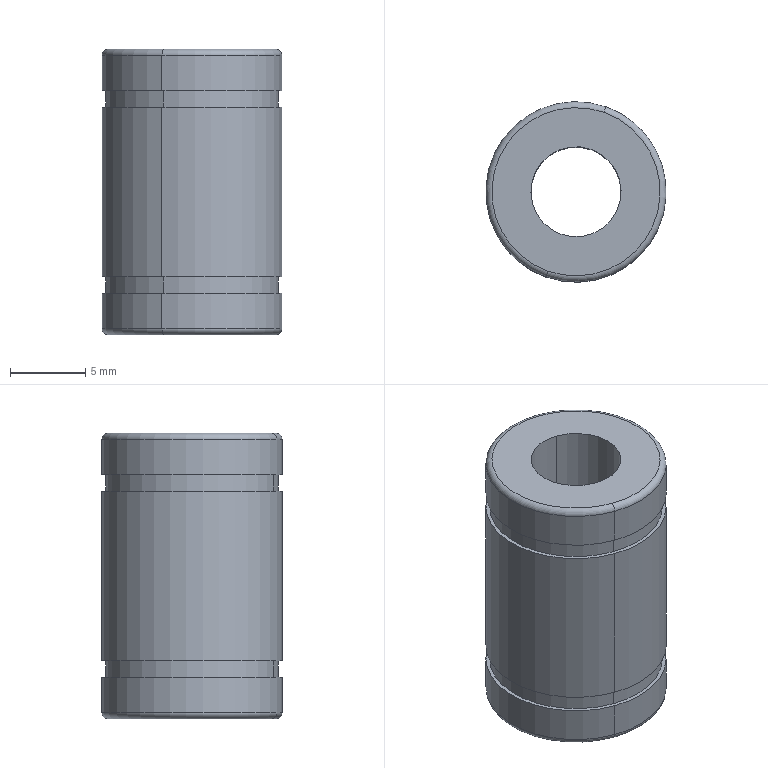Component | SolidWorks | LinearBearingMisumiLMU6-1 | 1 solid | 22 faces | box 12 x 12 x 19 mm | volume 1589 mm3 | cylinder 12 | plane 6 | torus 4 | commonest cylinder face diameters 12 x6 11.5 x4 6 x2 | material 45
build123d program:
from build123d import *


with BuildPart() as part:
    # Sketch1 → Revolve1 (revolve)
    with BuildSketch(Plane.XY, mode=Mode.PRIVATE) as revolve1_sk:
        with BuildLine():
            Line((0, 5.6), (0, 3))
            Line((0, 3), (19, 3))
            Line((19, 3), (19, 5.6))
            ThreePointArc((19, 5.6), (18.883, 5.883), (18.6, 6))
            Line((18.6, 6), (16.25, 6))
            Line((16.25, 6), (16.25, 5.75))
            Line((16.25, 5.75), (15.15, 5.75))
            Line((15.15, 5.75), (15.15, 6))
            Line((15.15, 6), (3.85, 6))
            Line((3.85, 6), (3.85, 5.75))
            Line((3.85, 5.75), (2.75, 5.75))
            Line((2.75, 5.75), (2.75, 6))
            Line((2.75, 6), (0.4, 6))
            ThreePointArc((0.4, 6), (0.1172, 5.883), (0, 5.6))
        make_face()
    revolve(revolve1_sk.sketch.rotate(Axis((19, 0, 0), (-1, 0, 0)), 270), axis=Axis((19, 0, 0), (-1, 0, 0)))


solid = part.part

# Placed as in the assembly
solid = solid.moved(Location((-10, 5.5, 13.5), (0, 90, 0)))
STEP:
#1=COLOUR_RGB('',0.7922,0.8196,0.9333);
#2=FILL_AREA_STYLE_COLOUR('',#1);
#3=FILL_AREA_STYLE('',(#2));
#4=SURFACE_STYLE_FILL_AREA(#3);
#5=SURFACE_SIDE_STYLE('',(#4));
#6=SURFACE_STYLE_USAGE(.BOTH.,#5);
#7=PRESENTATION_STYLE_ASSIGNMENT((#6));
#8=CARTESIAN_POINT('',(-0.315,0.4393,-0.1083));
#9=VERTEX_POINT('',#8);
#10=CARTESIAN_POINT('',(-0.4724,-0.006183,-0.1083));
#11=VERTEX_POINT('',#10);
#12=CARTESIAN_POINT('',(-0.3937,0.2165,-0.1083));
#13=DIRECTION('',(-0.,0.,-1.));
#14=DIRECTION('',(0.3332,0.9428,0.));
#15=AXIS2_PLACEMENT_3D('',#12,#13,#14);
#16=CIRCLE('',#15,0.2362);
#17=EDGE_CURVE('',#9,#11,#16,.T.);
#18=ORIENTED_EDGE('',*,*,#17,.T.);
#19=CARTESIAN_POINT('',(-0.4724,-0.006183,-0.2008));
#20=VERTEX_POINT('',#19);
#21=CARTESIAN_POINT('',(-0.4724,-0.006183,0.5315));
#22=DIRECTION('',(-0.,0.,-1.));
#23=VECTOR('',#22,39.37);
#24=LINE('',#21,#23);
#25=EDGE_CURVE('',#11,#20,#24,.T.);
#26=ORIENTED_EDGE('',*,*,#25,.T.);
#27=CARTESIAN_POINT('',(-0.315,0.4393,-0.2008));
#28=VERTEX_POINT('',#27);
#29=CARTESIAN_POINT('',(-0.3937,0.2165,-0.2008));
#30=DIRECTION('',(-0.,0.,-1.));
#31=DIRECTION('',(0.3332,0.9428,0.));
#32=AXIS2_PLACEMENT_3D('',#29,#30,#31);
#33=CIRCLE('',#32,0.2362);
#34=EDGE_CURVE('',#28,#20,#33,.T.);
#35=ORIENTED_EDGE('',*,*,#34,.F.);
#36=CARTESIAN_POINT('',(-0.315,0.4393,0.5315));
#37=DIRECTION('',(-0.,0.,-1.));
#38=VECTOR('',#37,39.37);
#39=LINE('',#36,#38);
#40=EDGE_CURVE('',#9,#28,#39,.T.);
#41=ORIENTED_EDGE('',*,*,#40,.F.);
#42=EDGE_LOOP('',(#18,#26,#35,#41));
#43=FACE_OUTER_BOUND('',#42,.T.);
#44=CARTESIAN_POINT('',(-0.3937,0.2165,0.5315));
#45=DIRECTION('',(-0.,0.,-1.));
#46=DIRECTION('',(0.3332,0.9428,0.));
#47=AXIS2_PLACEMENT_3D('',#44,#45,#46);
#48=CYLINDRICAL_SURFACE('',#47,0.2362);
#49=ADVANCED_FACE('',(#43),#48,.T.);
#50=CARTESIAN_POINT('',(-0.3183,0.43,-0.06496));
#51=VERTEX_POINT('',#50);
#52=CARTESIAN_POINT('',(-0.4691,0.003097,-0.06496));
#53=VERTEX_POINT('',#52);
#54=CARTESIAN_POINT('',(-0.3937,0.2165,-0.06496));
#55=DIRECTION('',(-0.,0.,-1.));
#56=DIRECTION('',(0.3332,0.9428,0.));
#57=AXIS2_PLACEMENT_3D('',#54,#55,#56);
#58=CIRCLE('',#57,0.2264);
#59=EDGE_CURVE('',#51,#53,#58,.T.);
#60=ORIENTED_EDGE('',*,*,#59,.T.);
#61=CARTESIAN_POINT('',(-0.4691,0.003097,-0.1083));
#62=VERTEX_POINT('',#61);
#63=CARTESIAN_POINT('',(-0.4691,0.003097,0.5315));
#64=DIRECTION('',(-0.,0.,-1.));
#65=VECTOR('',#64,39.37);
#66=LINE('',#63,#65);
#67=EDGE_CURVE('',#53,#62,#66,.T.);
#68=ORIENTED_EDGE('',*,*,#67,.T.);
#69=CARTESIAN_POINT('',(-0.3183,0.43,-0.1083));
#70=VERTEX_POINT('',#69);
#71=CARTESIAN_POINT('',(-0.3937,0.2165,-0.1083));
#72=DIRECTION('',(-0.,0.,-1.));
#73=DIRECTION('',(0.3332,0.9428,0.));
#74=AXIS2_PLACEMENT_3D('',#71,#72,#73);
#75=CIRCLE('',#74,0.2264);
#76=EDGE_CURVE('',#70,#62,#75,.T.);
#77=ORIENTED_EDGE('',*,*,#76,.F.);
#78=CARTESIAN_POINT('',(-0.3183,0.43,0.5315));
#79=DIRECTION('',(-0.,0.,-1.));
#80=VECTOR('',#79,39.37);
#81=LINE('',#78,#80);
#82=EDGE_CURVE('',#51,#70,#81,.T.);
#83=ORIENTED_EDGE('',*,*,#82,.F.);
#84=EDGE_LOOP('',(#60,#68,#77,#83));
#85=FACE_OUTER_BOUND('',#84,.T.);
#86=CARTESIAN_POINT('',(-0.3937,0.2165,0.5315));
#87=DIRECTION('',(-0.,0.,-1.));
#88=DIRECTION('',(0.3332,0.9428,0.));
#89=AXIS2_PLACEMENT_3D('',#86,#87,#88);
#90=CYLINDRICAL_SURFACE('',#89,0.2264);
#91=ADVANCED_FACE('',(#85),#90,.T.);
#92=CARTESIAN_POINT('',(-0.315,0.4393,0.3799));
#93=VERTEX_POINT('',#92);
#94=CARTESIAN_POINT('',(-0.4724,-0.006183,0.3799));
#95=VERTEX_POINT('',#94);
#96=CARTESIAN_POINT('',(-0.3937,0.2165,0.3799));
#97=DIRECTION('',(-0.,0.,-1.));
#98=DIRECTION('',(0.3332,0.9428,0.));
#99=AXIS2_PLACEMENT_3D('',#96,#97,#98);
#100=CIRCLE('',#99,0.2362);
#101=EDGE_CURVE('',#93,#95,#100,.T.);
#102=ORIENTED_EDGE('',*,*,#101,.T.);
#103=CARTESIAN_POINT('',(-0.4724,-0.006183,-0.06496));
#104=VERTEX_POINT('',#103);
#105=CARTESIAN_POINT('',(-0.4724,-0.006183,0.5315));
#106=DIRECTION('',(-0.,0.,-1.));
#107=VECTOR('',#106,39.37);
#108=LINE('',#105,#107);
#109=EDGE_CURVE('',#95,#104,#108,.T.);
#110=ORIENTED_EDGE('',*,*,#109,.T.);
#111=CARTESIAN_POINT('',(-0.315,0.4393,-0.06496));
#112=VERTEX_POINT('',#111);
#113=CARTESIAN_POINT('',(-0.3937,0.2165,-0.06496));
#114=DIRECTION('',(-0.,0.,-1.));
#115=DIRECTION('',(0.3332,0.9428,0.));
#116=AXIS2_PLACEMENT_3D('',#113,#114,#115);
#117=CIRCLE('',#116,0.2362);
#118=EDGE_CURVE('',#112,#104,#117,.T.);
#119=ORIENTED_EDGE('',*,*,#118,.F.);
#120=CARTESIAN_POINT('',(-0.315,0.4393,0.5315));
#121=DIRECTION('',(-0.,0.,-1.));
#122=VECTOR('',#121,39.37);
#123=LINE('',#120,#122);
#124=EDGE_CURVE('',#93,#112,#123,.T.);
#125=ORIENTED_EDGE('',*,*,#124,.F.);
#126=EDGE_LOOP('',(#102,#110,#119,#125));
#127=FACE_OUTER_BOUND('',#126,.T.);
#128=CARTESIAN_POINT('',(-0.3937,0.2165,0.5315));
#129=DIRECTION('',(-0.,0.,-1.));
#130=DIRECTION('',(0.3332,0.9428,0.));
#131=AXIS2_PLACEMENT_3D('',#128,#129,#130);
#132=CYLINDRICAL_SURFACE('',#131,0.2362);
#133=ADVANCED_FACE('',(#127),#132,.T.);
#134=CARTESIAN_POINT('',(-0.3183,0.43,0.4232));
#135=VERTEX_POINT('',#134);
#136=CARTESIAN_POINT('',(-0.4691,0.003097,0.4232));
#137=VERTEX_POINT('',#136);
#138=CARTESIAN_POINT('',(-0.3937,0.2165,0.4232));
#139=DIRECTION('',(-0.,0.,-1.));
#140=DIRECTION('',(0.3332,0.9428,0.));
#141=AXIS2_PLACEMENT_3D('',#138,#139,#140);
#142=CIRCLE('',#141,0.2264);
#143=EDGE_CURVE('',#135,#137,#142,.T.);
#144=ORIENTED_EDGE('',*,*,#143,.T.);
#145=CARTESIAN_POINT('',(-0.4691,0.003097,0.3799));
#146=VERTEX_POINT('',#145);
#147=CARTESIAN_POINT('',(-0.4691,0.003097,0.5315));
#148=DIRECTION('',(-0.,0.,-1.));
#149=VECTOR('',#148,39.37);
#150=LINE('',#147,#149);
#151=EDGE_CURVE('',#137,#146,#150,.T.);
#152=ORIENTED_EDGE('',*,*,#151,.T.);
#153=CARTESIAN_POINT('',(-0.3183,0.43,0.3799));
#154=VERTEX_POINT('',#153);
#155=CARTESIAN_POINT('',(-0.3937,0.2165,0.3799));
#156=DIRECTION('',(-0.,0.,-1.));
#157=DIRECTION('',(0.3332,0.9428,0.));
#158=AXIS2_PLACEMENT_3D('',#155,#156,#157);
#159=CIRCLE('',#158,0.2264);
#160=EDGE_CURVE('',#154,#146,#159,.T.);
#161=ORIENTED_EDGE('',*,*,#160,.F.);
#162=CARTESIAN_POINT('',(-0.3183,0.43,0.5315));
#163=DIRECTION('',(-0.,0.,-1.));
#164=VECTOR('',#163,39.37);
#165=LINE('',#162,#164);
#166=EDGE_CURVE('',#135,#154,#165,.T.);
#167=ORIENTED_EDGE('',*,*,#166,.F.);
#168=EDGE_LOOP('',(#144,#152,#161,#167));
#169=FACE_OUTER_BOUND('',#168,.T.);
#170=CARTESIAN_POINT('',(-0.3937,0.2165,0.5315));
#171=DIRECTION('',(-0.,0.,-1.));
#172=DIRECTION('',(0.3332,0.9428,0.));
#173=AXIS2_PLACEMENT_3D('',#170,#171,#172);
#174=CYLINDRICAL_SURFACE('',#173,0.2264);
#175=ADVANCED_FACE('',(#169),#174,.T.);
#176=CARTESIAN_POINT('',(-0.315,0.4393,0.5157));
#177=VERTEX_POINT('',#176);
#178=CARTESIAN_POINT('',(-0.4724,-0.006183,0.5157));
#179=VERTEX_POINT('',#178);
#180=CARTESIAN_POINT('',(-0.3937,0.2165,0.5157));
#181=DIRECTION('',(-0.,0.,-1.));
#182=DIRECTION('',(0.3332,0.9428,0.));
#183=AXIS2_PLACEMENT_3D('',#180,#181,#182);
#184=CIRCLE('',#183,0.2362);
#185=EDGE_CURVE('',#177,#179,#184,.T.);
#186=ORIENTED_EDGE('',*,*,#185,.T.);
#187=CARTESIAN_POINT('',(-0.4724,-0.006183,0.4232));
#188=VERTEX_POINT('',#187);
#189=CARTESIAN_POINT('',(-0.4724,-0.006183,0.5315));
#190=DIRECTION('',(-0.,0.,-1.));
#191=VECTOR('',#190,39.37);
#192=LINE('',#189,#191);
#193=EDGE_CURVE('',#179,#188,#192,.T.);
#194=ORIENTED_EDGE('',*,*,#193,.T.);
#195=CARTESIAN_POINT('',(-0.315,0.4393,0.4232));
#196=VERTEX_POINT('',#195);
#197=CARTESIAN_POINT('',(-0.3937,0.2165,0.4232));
#198=DIRECTION('',(-0.,0.,-1.));
#199=DIRECTION('',(0.3332,0.9428,0.));
#200=AXIS2_PLACEMENT_3D('',#197,#198,#199);
#201=CIRCLE('',#200,0.2362);
#202=EDGE_CURVE('',#196,#188,#201,.T.);
#203=ORIENTED_EDGE('',*,*,#202,.F.);
#204=CARTESIAN_POINT('',(-0.315,0.4393,0.5315));
#205=DIRECTION('',(-0.,0.,-1.));
#206=VECTOR('',#205,39.37);
#207=LINE('',#204,#206);
#208=EDGE_CURVE('',#177,#196,#207,.T.);
#209=ORIENTED_EDGE('',*,*,#208,.F.);
#210=EDGE_LOOP('',(#186,#194,#203,#209));
#211=FACE_OUTER_BOUND('',#210,.T.);
#212=CARTESIAN_POINT('',(-0.3937,0.2165,0.5315));
#213=DIRECTION('',(-0.,0.,-1.));
#214=DIRECTION('',(0.3332,0.9428,0.));
#215=AXIS2_PLACEMENT_3D('',#212,#213,#214);
#216=CYLINDRICAL_SURFACE('',#215,0.2362);
#217=ADVANCED_FACE('',(#211),#216,.T.);
#218=CARTESIAN_POINT('',(-0.3202,0.4244,0.5315));
#219=VERTEX_POINT('',#218);
#220=CARTESIAN_POINT('',(-0.4672,0.008665,0.5315));
#221=VERTEX_POINT('',#220);
#222=CARTESIAN_POINT('',(-0.3937,0.2165,0.5315));
#223=DIRECTION('',(-0.,0.,-1.));
#224=DIRECTION('',(0.3332,0.9428,0.));
#225=AXIS2_PLACEMENT_3D('',#222,#223,#224);
#226=CIRCLE('',#225,0.2205);
#227=EDGE_CURVE('',#219,#221,#226,.T.);
#228=ORIENTED_EDGE('',*,*,#227,.T.);
#229=CARTESIAN_POINT('',(-0.4672,0.008665,0.5157));
#230=DIRECTION('',(0.9428,-0.3332,-0.));
#231=DIRECTION('',(0.3332,0.9428,0.));
#232=AXIS2_PLACEMENT_3D('',#229,#230,#231);
#233=CIRCLE('',#232,0.01575);
#234=EDGE_CURVE('',#221,#179,#233,.T.);
#235=ORIENTED_EDGE('',*,*,#234,.T.);
#236=ORIENTED_EDGE('',*,*,#185,.F.);
#237=CARTESIAN_POINT('',(-0.3202,0.4244,0.5157));
#238=DIRECTION('',(-0.9428,0.3332,0.));
#239=DIRECTION('',(-0.3332,-0.9428,0.));
#240=AXIS2_PLACEMENT_3D('',#237,#238,#239);
#241=CIRCLE('',#240,0.01575);
#242=EDGE_CURVE('',#219,#177,#241,.T.);
#243=ORIENTED_EDGE('',*,*,#242,.F.);
#244=EDGE_LOOP('',(#228,#235,#236,#243));
#245=FACE_OUTER_BOUND('',#244,.T.);
#246=CARTESIAN_POINT('',(-0.3937,0.2165,0.5157));
#247=DIRECTION('',(-0.,0.,-1.));
#248=DIRECTION('',(0.3332,0.9428,0.));
#249=AXIS2_PLACEMENT_3D('',#246,#247,#248);
#250=TOROIDAL_SURFACE('',#249,0.2205,0.01575);
#251=ADVANCED_FACE('',(#245),#250,.T.);
#252=CARTESIAN_POINT('',(-0.4331,0.1052,0.5315));
#253=VERTEX_POINT('',#252);
#254=CARTESIAN_POINT('',(-0.3543,0.3279,0.5315));
#255=VERTEX_POINT('',#254);
#256=CARTESIAN_POINT('',(-0.3937,0.2165,0.5315));
#257=DIRECTION('',(-0.,0.,-1.));
#258=DIRECTION('',(0.3332,0.9428,0.));
#259=AXIS2_PLACEMENT_3D('',#256,#257,#258);
#260=CIRCLE('',#259,0.1181);
#261=EDGE_CURVE('',#253,#255,#260,.T.);
#262=ORIENTED_EDGE('',*,*,#261,.F.);
#263=CARTESIAN_POINT('',(-0.4331,0.1052,-0.2165));
#264=VERTEX_POINT('',#263);
#265=CARTESIAN_POINT('',(-0.4331,0.1052,0.5315));
#266=DIRECTION('',(-0.,0.,-1.));
#267=VECTOR('',#266,39.37);
#268=LINE('',#265,#267);
#269=EDGE_CURVE('',#253,#264,#268,.T.);
#270=ORIENTED_EDGE('',*,*,#269,.T.);
#271=CARTESIAN_POINT('',(-0.3543,0.3279,-0.2165));
#272=VERTEX_POINT('',#271);
#273=CARTESIAN_POINT('',(-0.3937,0.2165,-0.2165));
#274=DIRECTION('',(-0.,0.,-1.));
#275=DIRECTION('',(0.3332,0.9428,0.));
#276=AXIS2_PLACEMENT_3D('',#273,#274,#275);
#277=CIRCLE('',#276,0.1181);
#278=EDGE_CURVE('',#264,#272,#277,.T.);
#279=ORIENTED_EDGE('',*,*,#278,.T.);
#280=CARTESIAN_POINT('',(-0.3543,0.3279,0.5315));
#281=DIRECTION('',(-0.,0.,-1.));
#282=VECTOR('',#281,39.37);
#283=LINE('',#280,#282);
#284=EDGE_CURVE('',#255,#272,#283,.T.);
#285=ORIENTED_EDGE('',*,*,#284,.F.);
#286=EDGE_LOOP('',(#262,#270,#279,#285));
#287=FACE_OUTER_BOUND('',#286,.T.);
#288=CARTESIAN_POINT('',(-0.3937,0.2165,0.5315));
#289=DIRECTION('',(-0.,0.,-1.));
#290=DIRECTION('',(0.3332,0.9428,0.));
#291=AXIS2_PLACEMENT_3D('',#288,#289,#290);
#292=CYLINDRICAL_SURFACE('',#291,0.1181);
#293=ADVANCED_FACE('',(#287),#292,.F.);
#294=ORIENTED_EDGE('',*,*,#34,.T.);
#295=CARTESIAN_POINT('',(-0.4672,0.008665,-0.2165));
#296=VERTEX_POINT('',#295);
#297=CARTESIAN_POINT('',(-0.4672,0.008665,-0.2008));
#298=DIRECTION('',(0.9428,-0.3332,-0.));
#299=DIRECTION('',(0.3332,0.9428,0.));
#300=AXIS2_PLACEMENT_3D('',#297,#298,#299);
#301=CIRCLE('',#300,0.01575);
#302=EDGE_CURVE('',#20,#296,#301,.T.);
#303=ORIENTED_EDGE('',*,*,#302,.T.);
#304=CARTESIAN_POINT('',(-0.3202,0.4244,-0.2165));
#305=VERTEX_POINT('',#304);
#306=CARTESIAN_POINT('',(-0.3937,0.2165,-0.2165));
#307=DIRECTION('',(-0.,0.,-1.));
#308=DIRECTION('',(0.3332,0.9428,0.));
#309=AXIS2_PLACEMENT_3D('',#306,#307,#308);
#310=CIRCLE('',#309,0.2205);
#311=EDGE_CURVE('',#305,#296,#310,.T.);
#312=ORIENTED_EDGE('',*,*,#311,.F.);
#313=CARTESIAN_POINT('',(-0.3202,0.4244,-0.2008));
#314=DIRECTION('',(-0.9428,0.3332,0.));
#315=DIRECTION('',(-0.3332,-0.9428,0.));
#316=AXIS2_PLACEMENT_3D('',#313,#314,#315);
#317=CIRCLE('',#316,0.01575);
#318=EDGE_CURVE('',#28,#305,#317,.T.);
#319=ORIENTED_EDGE('',*,*,#318,.F.);
#320=EDGE_LOOP('',(#294,#303,#312,#319));
#321=FACE_OUTER_BOUND('',#320,.T.);
#322=CARTESIAN_POINT('',(-0.3937,0.2165,-0.2008));
#323=DIRECTION('',(-0.,0.,-1.));
#324=DIRECTION('',(0.3332,0.9428,0.));
#325=AXIS2_PLACEMENT_3D('',#322,#323,#324);
#326=TOROIDAL_SURFACE('',#325,0.2205,0.01575);
#327=ADVANCED_FACE('',(#321),#326,.T.);
#328=ORIENTED_EDGE('',*,*,#302,.F.);
#329=CARTESIAN_POINT('',(-0.3937,0.2165,-0.2008));
#330=DIRECTION('',(-0.,0.,-1.));
#331=DIRECTION('',(0.3332,0.9428,0.));
#332=AXIS2_PLACEMENT_3D('',#329,#330,#331);
#333=CIRCLE('',#332,0.2362);
#334=EDGE_CURVE('',#20,#28,#333,.T.);
#335=ORIENTED_EDGE('',*,*,#334,.T.);
#336=ORIENTED_EDGE('',*,*,#318,.T.);
#337=CARTESIAN_POINT('',(-0.3937,0.2165,-0.2165));
#338=DIRECTION('',(-0.,0.,-1.));
#339=DIRECTION('',(0.3332,0.9428,0.));
#340=AXIS2_PLACEMENT_3D('',#337,#338,#339);
#341=CIRCLE('',#340,0.2205);
#342=EDGE_CURVE('',#296,#305,#341,.T.);
#343=ORIENTED_EDGE('',*,*,#342,.F.);
#344=EDGE_LOOP('',(#328,#335,#336,#343));
#345=FACE_OUTER_BOUND('',#344,.T.);
#346=CARTESIAN_POINT('',(-0.3937,0.2165,-0.2008));
#347=DIRECTION('',(-0.,0.,-1.));
#348=DIRECTION('',(0.3332,0.9428,0.));
#349=AXIS2_PLACEMENT_3D('',#346,#347,#348);
#350=TOROIDAL_SURFACE('',#349,0.2205,0.01575);
#351=ADVANCED_FACE('',(#345),#350,.T.);
#352=CARTESIAN_POINT('',(-0.3937,0.2165,-0.2165));
#353=DIRECTION('',(-0.,0.,-1.));
#354=DIRECTION('',(0.3332,0.9428,0.));
#355=AXIS2_PLACEMENT_3D('',#352,#353,#354);
#356=CIRCLE('',#355,0.1181);
#357=EDGE_CURVE('',#272,#264,#356,.T.);
#358=ORIENTED_EDGE('',*,*,#357,.F.);
#359=ORIENTED_EDGE('',*,*,#278,.F.);
#360=EDGE_LOOP('',(#358,#359));
#361=FACE_BOUND('',#360,.T.);
#362=ORIENTED_EDGE('',*,*,#311,.T.);
#363=ORIENTED_EDGE('',*,*,#342,.T.);
#364=EDGE_LOOP('',(#362,#363));
#365=FACE_OUTER_BOUND('',#364,.T.);
#366=CARTESIAN_POINT('',(-0.1858,0.1431,-0.2165));
#367=DIRECTION('',(0.,-0.,1.));
#368=DIRECTION('',(-0.3332,-0.9428,-0.));
#369=AXIS2_PLACEMENT_3D('',#366,#367,#368);
#370=PLANE('',#369);
#371=ADVANCED_FACE('',(#361,#365),#370,.F.);
#372=ORIENTED_EDGE('',*,*,#269,.F.);
#373=CARTESIAN_POINT('',(-0.3937,0.2165,0.5315));
#374=DIRECTION('',(-0.,0.,-1.));
#375=DIRECTION('',(0.3332,0.9428,0.));
#376=AXIS2_PLACEMENT_3D('',#373,#374,#375);
#377=CIRCLE('',#376,0.1181);
#378=EDGE_CURVE('',#255,#253,#377,.T.);
#379=ORIENTED_EDGE('',*,*,#378,.F.);
#380=ORIENTED_EDGE('',*,*,#284,.T.);
#381=ORIENTED_EDGE('',*,*,#357,.T.);
#382=EDGE_LOOP('',(#372,#379,#380,#381));
#383=FACE_OUTER_BOUND('',#382,.T.);
#384=CARTESIAN_POINT('',(-0.3937,0.2165,0.5315));
#385=DIRECTION('',(-0.,0.,-1.));
#386=DIRECTION('',(0.3332,0.9428,0.));
#387=AXIS2_PLACEMENT_3D('',#384,#385,#386);
#388=CYLINDRICAL_SURFACE('',#387,0.1181);
#389=ADVANCED_FACE('',(#383),#388,.F.);
#390=ORIENTED_EDGE('',*,*,#227,.F.);
#391=CARTESIAN_POINT('',(-0.3937,0.2165,0.5315));
#392=DIRECTION('',(-0.,0.,-1.));
#393=DIRECTION('',(0.3332,0.9428,0.));
#394=AXIS2_PLACEMENT_3D('',#391,#392,#393);
#395=CIRCLE('',#394,0.2205);
#396=EDGE_CURVE('',#221,#219,#395,.T.);
#397=ORIENTED_EDGE('',*,*,#396,.F.);
#398=EDGE_LOOP('',(#390,#397));
#399=FACE_OUTER_BOUND('',#398,.T.);
#400=ORIENTED_EDGE('',*,*,#378,.T.);
#401=ORIENTED_EDGE('',*,*,#261,.T.);
#402=EDGE_LOOP('',(#400,#401));
#403=FACE_BOUND('',#402,.T.);
#404=CARTESIAN_POINT('',(-0.2823,0.1772,0.5315));
#405=DIRECTION('',(-0.,0.,-1.));
#406=DIRECTION('',(0.3332,0.9428,0.));
#407=AXIS2_PLACEMENT_3D('',#404,#405,#406);
#408=PLANE('',#407);
#409=ADVANCED_FACE('',(#399,#403),#408,.F.);
#410=ORIENTED_EDGE('',*,*,#234,.F.);
#411=ORIENTED_EDGE('',*,*,#396,.T.);
#412=ORIENTED_EDGE('',*,*,#242,.T.);
#413=CARTESIAN_POINT('',(-0.3937,0.2165,0.5157));
#414=DIRECTION('',(-0.,0.,-1.));
#415=DIRECTION('',(0.3332,0.9428,0.));
#416=AXIS2_PLACEMENT_3D('',#413,#414,#415);
#417=CIRCLE('',#416,0.2362);
#418=EDGE_CURVE('',#179,#177,#417,.T.);
#419=ORIENTED_EDGE('',*,*,#418,.F.);
#420=EDGE_LOOP('',(#410,#411,#412,#419));
#421=FACE_OUTER_BOUND('',#420,.T.);
#422=CARTESIAN_POINT('',(-0.3937,0.2165,0.5157));
#423=DIRECTION('',(-0.,0.,-1.));
#424=DIRECTION('',(0.3332,0.9428,0.));
#425=AXIS2_PLACEMENT_3D('',#422,#423,#424);
#426=TOROIDAL_SURFACE('',#425,0.2205,0.01575);
#427=ADVANCED_FACE('',(#421),#426,.T.);
#428=ORIENTED_EDGE('',*,*,#193,.F.);
#429=ORIENTED_EDGE('',*,*,#418,.T.);
#430=ORIENTED_EDGE('',*,*,#208,.T.);
#431=CARTESIAN_POINT('',(-0.3937,0.2165,0.4232));
#432=DIRECTION('',(-0.,0.,-1.));
#433=DIRECTION('',(0.3332,0.9428,0.));
#434=AXIS2_PLACEMENT_3D('',#431,#432,#433);
#435=CIRCLE('',#434,0.2362);
#436=EDGE_CURVE('',#188,#196,#435,.T.);
#437=ORIENTED_EDGE('',*,*,#436,.F.);
#438=EDGE_LOOP('',(#428,#429,#430,#437));
#439=FACE_OUTER_BOUND('',#438,.T.);
#440=CARTESIAN_POINT('',(-0.3937,0.2165,0.5315));
#441=DIRECTION('',(-0.,0.,-1.));
#442=DIRECTION('',(0.3332,0.9428,0.));
#443=AXIS2_PLACEMENT_3D('',#440,#441,#442);
#444=CYLINDRICAL_SURFACE('',#443,0.2362);
#445=ADVANCED_FACE('',(#439),#444,.T.);
#446=ORIENTED_EDGE('',*,*,#143,.F.);
#447=CARTESIAN_POINT('',(-0.3937,0.2165,0.4232));
#448=DIRECTION('',(-0.,0.,-1.));
#449=DIRECTION('',(0.3332,0.9428,0.));
#450=AXIS2_PLACEMENT_3D('',#447,#448,#449);
#451=CIRCLE('',#450,0.2264);
#452=EDGE_CURVE('',#137,#135,#451,.T.);
#453=ORIENTED_EDGE('',*,*,#452,.F.);
#454=EDGE_LOOP('',(#446,#453));
#455=FACE_BOUND('',#454,.T.);
#456=ORIENTED_EDGE('',*,*,#202,.T.);
#457=ORIENTED_EDGE('',*,*,#436,.T.);
#458=EDGE_LOOP('',(#456,#457));
#459=FACE_OUTER_BOUND('',#458,.T.);
#460=CARTESIAN_POINT('',(-0.171,0.1378,0.4232));
#461=DIRECTION('',(0.,-0.,1.));
#462=DIRECTION('',(-0.3332,-0.9428,-0.));
#463=AXIS2_PLACEMENT_3D('',#460,#461,#462);
#464=PLANE('',#463);
#465=ADVANCED_FACE('',(#455,#459),#464,.F.);
#466=ORIENTED_EDGE('',*,*,#151,.F.);
#467=ORIENTED_EDGE('',*,*,#452,.T.);
#468=ORIENTED_EDGE('',*,*,#166,.T.);
#469=CARTESIAN_POINT('',(-0.3937,0.2165,0.3799));
#470=DIRECTION('',(-0.,0.,-1.));
#471=DIRECTION('',(0.3332,0.9428,0.));
#472=AXIS2_PLACEMENT_3D('',#469,#470,#471);
#473=CIRCLE('',#472,0.2264);
#474=EDGE_CURVE('',#146,#154,#473,.T.);
#475=ORIENTED_EDGE('',*,*,#474,.F.);
#476=EDGE_LOOP('',(#466,#467,#468,#475));
#477=FACE_OUTER_BOUND('',#476,.T.);
#478=CARTESIAN_POINT('',(-0.3937,0.2165,0.5315));
#479=DIRECTION('',(-0.,0.,-1.));
#480=DIRECTION('',(0.3332,0.9428,0.));
#481=AXIS2_PLACEMENT_3D('',#478,#479,#480);
#482=CYLINDRICAL_SURFACE('',#481,0.2264);
#483=ADVANCED_FACE('',(#477),#482,.T.);
#484=ORIENTED_EDGE('',*,*,#101,.F.);
#485=CARTESIAN_POINT('',(-0.3937,0.2165,0.3799));
#486=DIRECTION('',(-0.,0.,-1.));
#487=DIRECTION('',(0.3332,0.9428,0.));
#488=AXIS2_PLACEMENT_3D('',#485,#486,#487);
#489=CIRCLE('',#488,0.2362);
#490=EDGE_CURVE('',#95,#93,#489,.T.);
#491=ORIENTED_EDGE('',*,*,#490,.F.);
#492=EDGE_LOOP('',(#484,#491));
#493=FACE_OUTER_BOUND('',#492,.T.);
#494=ORIENTED_EDGE('',*,*,#160,.T.);
#495=ORIENTED_EDGE('',*,*,#474,.T.);
#496=EDGE_LOOP('',(#494,#495));
#497=FACE_BOUND('',#496,.T.);
#498=CARTESIAN_POINT('',(-0.1803,0.1411,0.3799));
#499=DIRECTION('',(-0.,0.,-1.));
#500=DIRECTION('',(0.3332,0.9428,0.));
#501=AXIS2_PLACEMENT_3D('',#498,#499,#500);
#502=PLANE('',#501);
#503=ADVANCED_FACE('',(#493,#497),#502,.F.);
#504=ORIENTED_EDGE('',*,*,#109,.F.);
#505=ORIENTED_EDGE('',*,*,#490,.T.);
#506=ORIENTED_EDGE('',*,*,#124,.T.);
#507=CARTESIAN_POINT('',(-0.3937,0.2165,-0.06496));
#508=DIRECTION('',(-0.,0.,-1.));
#509=DIRECTION('',(0.3332,0.9428,0.));
#510=AXIS2_PLACEMENT_3D('',#507,#508,#509);
#511=CIRCLE('',#510,0.2362);
#512=EDGE_CURVE('',#104,#112,#511,.T.);
#513=ORIENTED_EDGE('',*,*,#512,.F.);
#514=EDGE_LOOP('',(#504,#505,#506,#513));
#515=FACE_OUTER_BOUND('',#514,.T.);
#516=CARTESIAN_POINT('',(-0.3937,0.2165,0.5315));
#517=DIRECTION('',(-0.,0.,-1.));
#518=DIRECTION('',(0.3332,0.9428,0.));
#519=AXIS2_PLACEMENT_3D('',#516,#517,#518);
#520=CYLINDRICAL_SURFACE('',#519,0.2362);
#521=ADVANCED_FACE('',(#515),#520,.T.);
#522=ORIENTED_EDGE('',*,*,#59,.F.);
#523=CARTESIAN_POINT('',(-0.3937,0.2165,-0.06496));
#524=DIRECTION('',(-0.,0.,-1.));
#525=DIRECTION('',(0.3332,0.9428,0.));
#526=AXIS2_PLACEMENT_3D('',#523,#524,#525);
#527=CIRCLE('',#526,0.2264);
#528=EDGE_CURVE('',#53,#51,#527,.T.);
#529=ORIENTED_EDGE('',*,*,#528,.F.);
#530=EDGE_LOOP('',(#522,#529));
#531=FACE_BOUND('',#530,.T.);
#532=ORIENTED_EDGE('',*,*,#118,.T.);
#533=ORIENTED_EDGE('',*,*,#512,.T.);
#534=EDGE_LOOP('',(#532,#533));
#535=FACE_OUTER_BOUND('',#534,.T.);
#536=CARTESIAN_POINT('',(-0.171,0.1378,-0.06496));
#537=DIRECTION('',(0.,-0.,1.));
#538=DIRECTION('',(-0.3332,-0.9428,-0.));
#539=AXIS2_PLACEMENT_3D('',#536,#537,#538);
#540=PLANE('',#539);
#541=ADVANCED_FACE('',(#531,#535),#540,.F.);
#542=ORIENTED_EDGE('',*,*,#67,.F.);
#543=ORIENTED_EDGE('',*,*,#528,.T.);
#544=ORIENTED_EDGE('',*,*,#82,.T.);
#545=CARTESIAN_POINT('',(-0.3937,0.2165,-0.1083));
#546=DIRECTION('',(-0.,0.,-1.));
#547=DIRECTION('',(0.3332,0.9428,0.));
#548=AXIS2_PLACEMENT_3D('',#545,#546,#547);
#549=CIRCLE('',#548,0.2264);
#550=EDGE_CURVE('',#62,#70,#549,.T.);
#551=ORIENTED_EDGE('',*,*,#550,.F.);
#552=EDGE_LOOP('',(#542,#543,#544,#551));
#553=FACE_OUTER_BOUND('',#552,.T.);
#554=CARTESIAN_POINT('',(-0.3937,0.2165,0.5315));
#555=DIRECTION('',(-0.,0.,-1.));
#556=DIRECTION('',(0.3332,0.9428,0.));
#557=AXIS2_PLACEMENT_3D('',#554,#555,#556);
#558=CYLINDRICAL_SURFACE('',#557,0.2264);
#559=ADVANCED_FACE('',(#553),#558,.T.);
#560=ORIENTED_EDGE('',*,*,#17,.F.);
#561=CARTESIAN_POINT('',(-0.3937,0.2165,-0.1083));
#562=DIRECTION('',(-0.,0.,-1.));
#563=DIRECTION('',(0.3332,0.9428,0.));
#564=AXIS2_PLACEMENT_3D('',#561,#562,#563);
#565=CIRCLE('',#564,0.2362);
#566=EDGE_CURVE('',#11,#9,#565,.T.);
#567=ORIENTED_EDGE('',*,*,#566,.F.);
#568=EDGE_LOOP('',(#560,#567));
#569=FACE_OUTER_BOUND('',#568,.T.);
#570=ORIENTED_EDGE('',*,*,#76,.T.);
#571=ORIENTED_EDGE('',*,*,#550,.T.);
#572=EDGE_LOOP('',(#570,#571));
#573=FACE_BOUND('',#572,.T.);
#574=CARTESIAN_POINT('',(-0.1803,0.1411,-0.1083));
#575=DIRECTION('',(-0.,0.,-1.));
#576=DIRECTION('',(0.3332,0.9428,0.));
#577=AXIS2_PLACEMENT_3D('',#574,#575,#576);
#578=PLANE('',#577);
#579=ADVANCED_FACE('',(#569,#573),#578,.F.);
#580=ORIENTED_EDGE('',*,*,#25,.F.);
#581=ORIENTED_EDGE('',*,*,#566,.T.);
#582=ORIENTED_EDGE('',*,*,#40,.T.);
#583=ORIENTED_EDGE('',*,*,#334,.F.);
#584=EDGE_LOOP('',(#580,#581,#582,#583));
#585=FACE_OUTER_BOUND('',#584,.T.);
#586=CARTESIAN_POINT('',(-0.3937,0.2165,0.5315));
#587=DIRECTION('',(-0.,0.,-1.));
#588=DIRECTION('',(0.3332,0.9428,0.));
#589=AXIS2_PLACEMENT_3D('',#586,#587,#588);
#590=CYLINDRICAL_SURFACE('',#589,0.2362);
#591=ADVANCED_FACE('',(#585),#590,.T.);
#592=CLOSED_SHELL('',(#49,#91,#133,#175,#217,#251,#293,#327,#351,#371,#389,#409,#427,#445,#465,#483,#503,#521,#541,#559,#579,#591));
#593=MANIFOLD_SOLID_BREP('',#592);
#594=STYLED_ITEM('',(#7),#593);
#595=(LENGTH_UNIT()NAMED_UNIT(*)SI_UNIT($,.METRE.));
#596=LENGTH_MEASURE_WITH_UNIT(LENGTH_MEASURE(0.0254),#595);
#597=DIMENSIONAL_EXPONENTS(1.,0.,0.,0.,0.,0.,0.);
#598=(CONVERSION_BASED_UNIT('',#596)LENGTH_UNIT()NAMED_UNIT(#597));
#599=UNCERTAINTY_MEASURE_WITH_UNIT(LENGTH_MEASURE(0.00001),#598,'','');
#600=(NAMED_UNIT(*)PLANE_ANGLE_UNIT()SI_UNIT($,.RADIAN.));
#601=(NAMED_UNIT(*)SI_UNIT($,.STERADIAN.)SOLID_ANGLE_UNIT());
#602=(GEOMETRIC_REPRESENTATION_CONTEXT(3)GLOBAL_UNCERTAINTY_ASSIGNED_CONTEXT((#599))GLOBAL_UNIT_ASSIGNED_CONTEXT((#598,#600,#601))REPRESENTATION_CONTEXT('',''));
#603=MECHANICAL_DESIGN_GEOMETRIC_PRESENTATION_REPRESENTATION('',(#594),#602);
#604=PRESENTATION_LAYER_ASSIGNMENT('','',(#594));
#605=CARTESIAN_POINT('',(0.,0.,0.));
#606=DIRECTION('',(0.,0.,1.));
#607=DIRECTION('',(1.,0.,0.));
#608=AXIS2_PLACEMENT_3D('',#605,#606,#607);
#609=(LENGTH_UNIT()NAMED_UNIT(*)SI_UNIT($,.METRE.));
#610=LENGTH_MEASURE_WITH_UNIT(LENGTH_MEASURE(0.0254),#609);
#611=DIMENSIONAL_EXPONENTS(1.,0.,0.,0.,0.,0.,0.);
#612=(CONVERSION_BASED_UNIT('',#610)LENGTH_UNIT()NAMED_UNIT(#611));
#613=UNCERTAINTY_MEASURE_WITH_UNIT(LENGTH_MEASURE(0.00001),#612,'','');
#614=(NAMED_UNIT(*)PLANE_ANGLE_UNIT()SI_UNIT($,.RADIAN.));
#615=(NAMED_UNIT(*)SI_UNIT($,.STERADIAN.)SOLID_ANGLE_UNIT());
#616=(GEOMETRIC_REPRESENTATION_CONTEXT(3)GLOBAL_UNCERTAINTY_ASSIGNED_CONTEXT((#613))GLOBAL_UNIT_ASSIGNED_CONTEXT((#612,#614,#615))REPRESENTATION_CONTEXT('',''));
#617=ADVANCED_BREP_SHAPE_REPRESENTATION('',(#593,#608),#616);